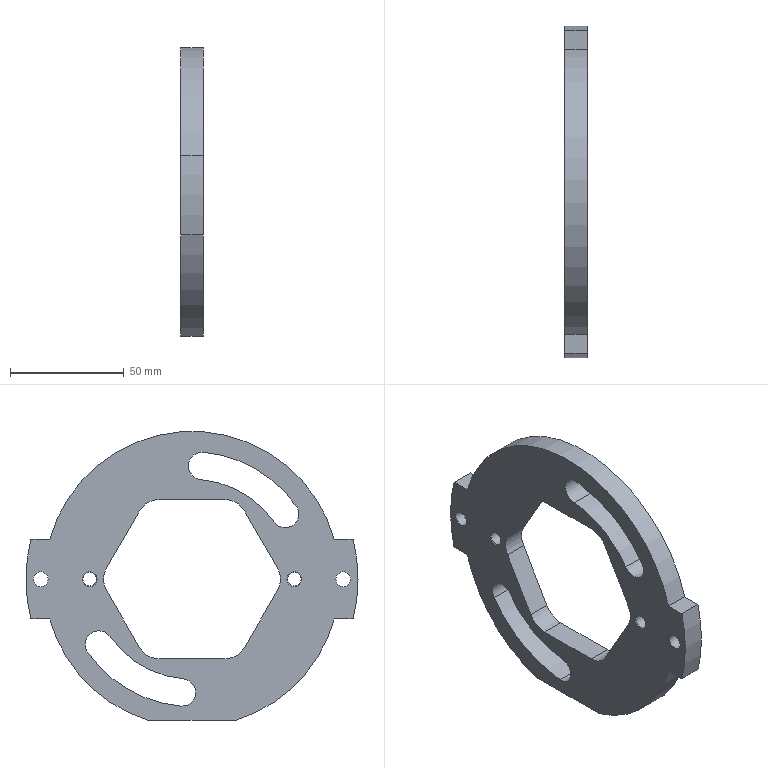Component | NX | HOUSING_COVER | 1 solid | 40 faces | volume 81531 mm3 | cylinder 23 | plane 13 | cone 4 | commonest cylinder face diameters 20 x6 12 x4 130 x3 88 x2 146 x2 112 x2 6 x2 6.5 x2